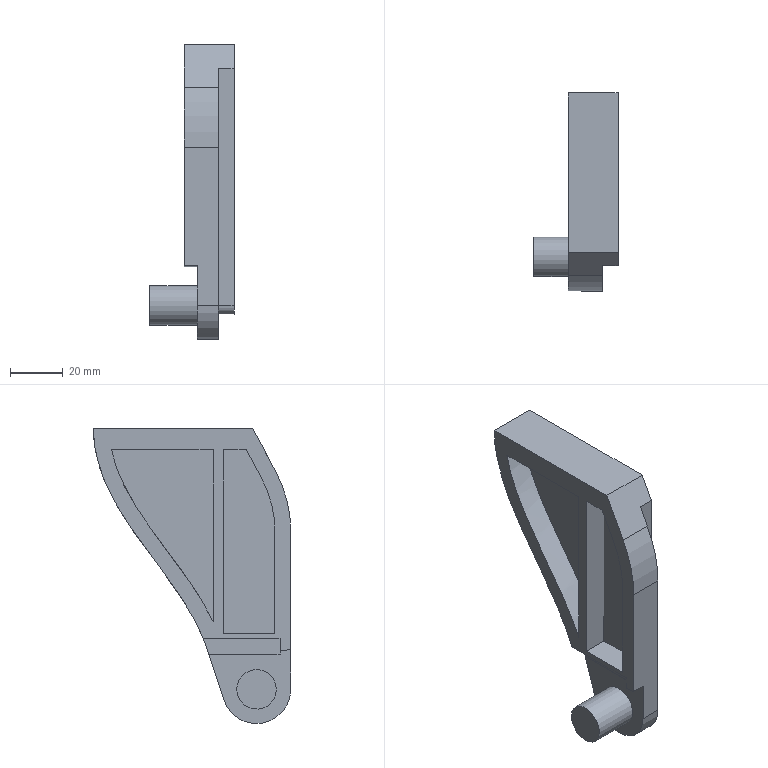Component | NX | TILT_BASE_ACC_2 | 1 solid | 35 faces | volume 48995 mm3 | plane 27 | cylinder 5 | other 3 | commonest cylinder face diameters 96 x1 26 x1 15 x1 84 x1 7 x1